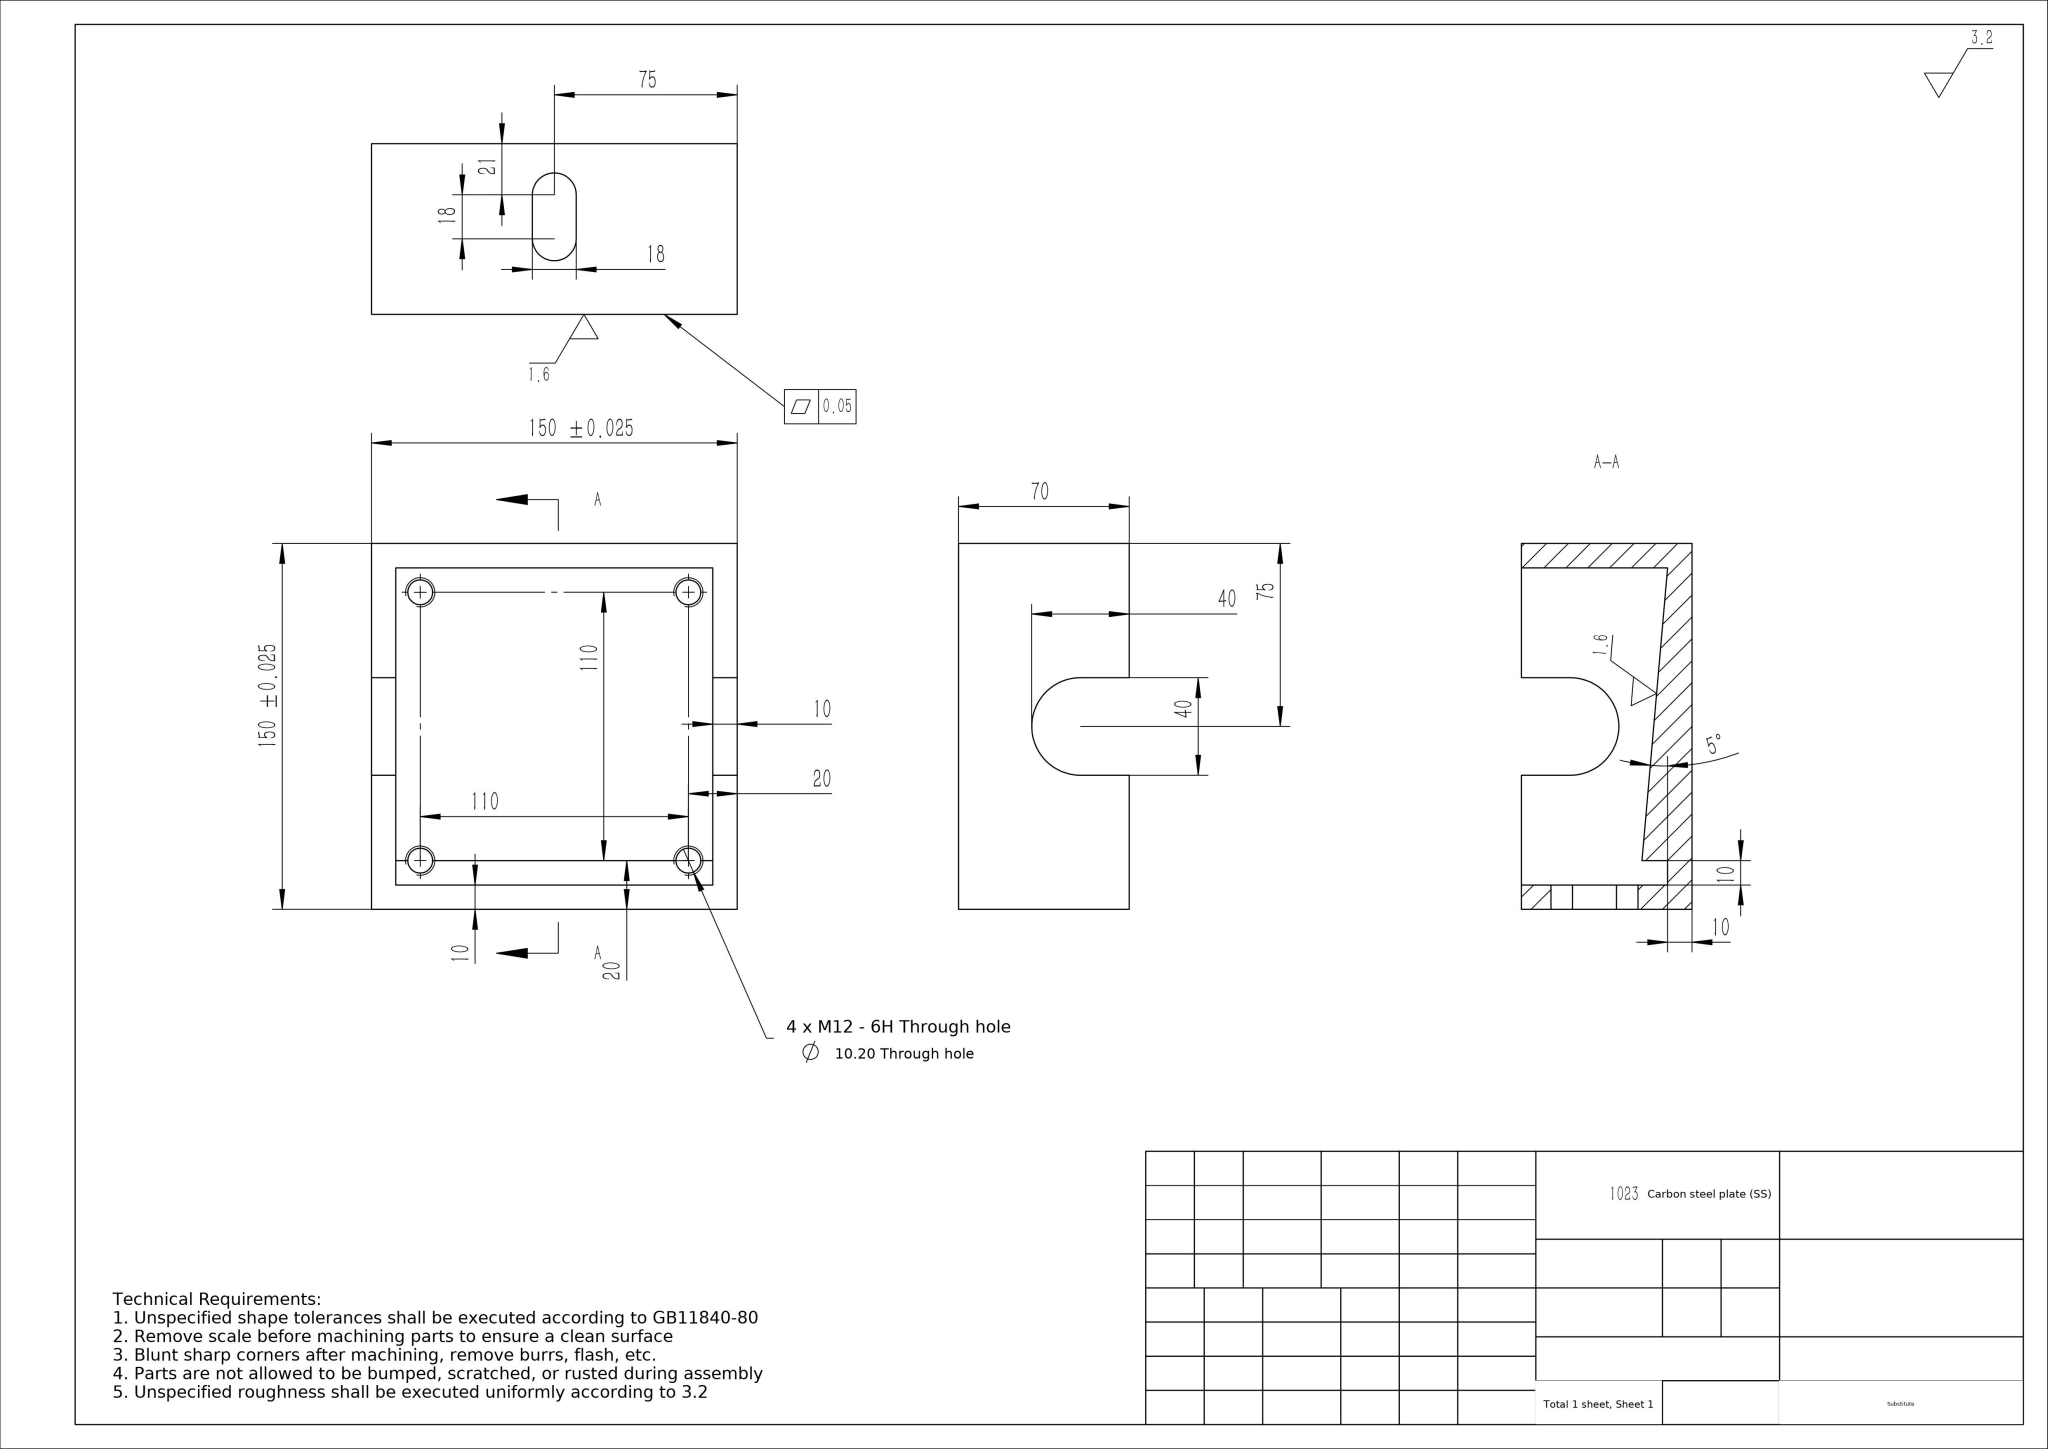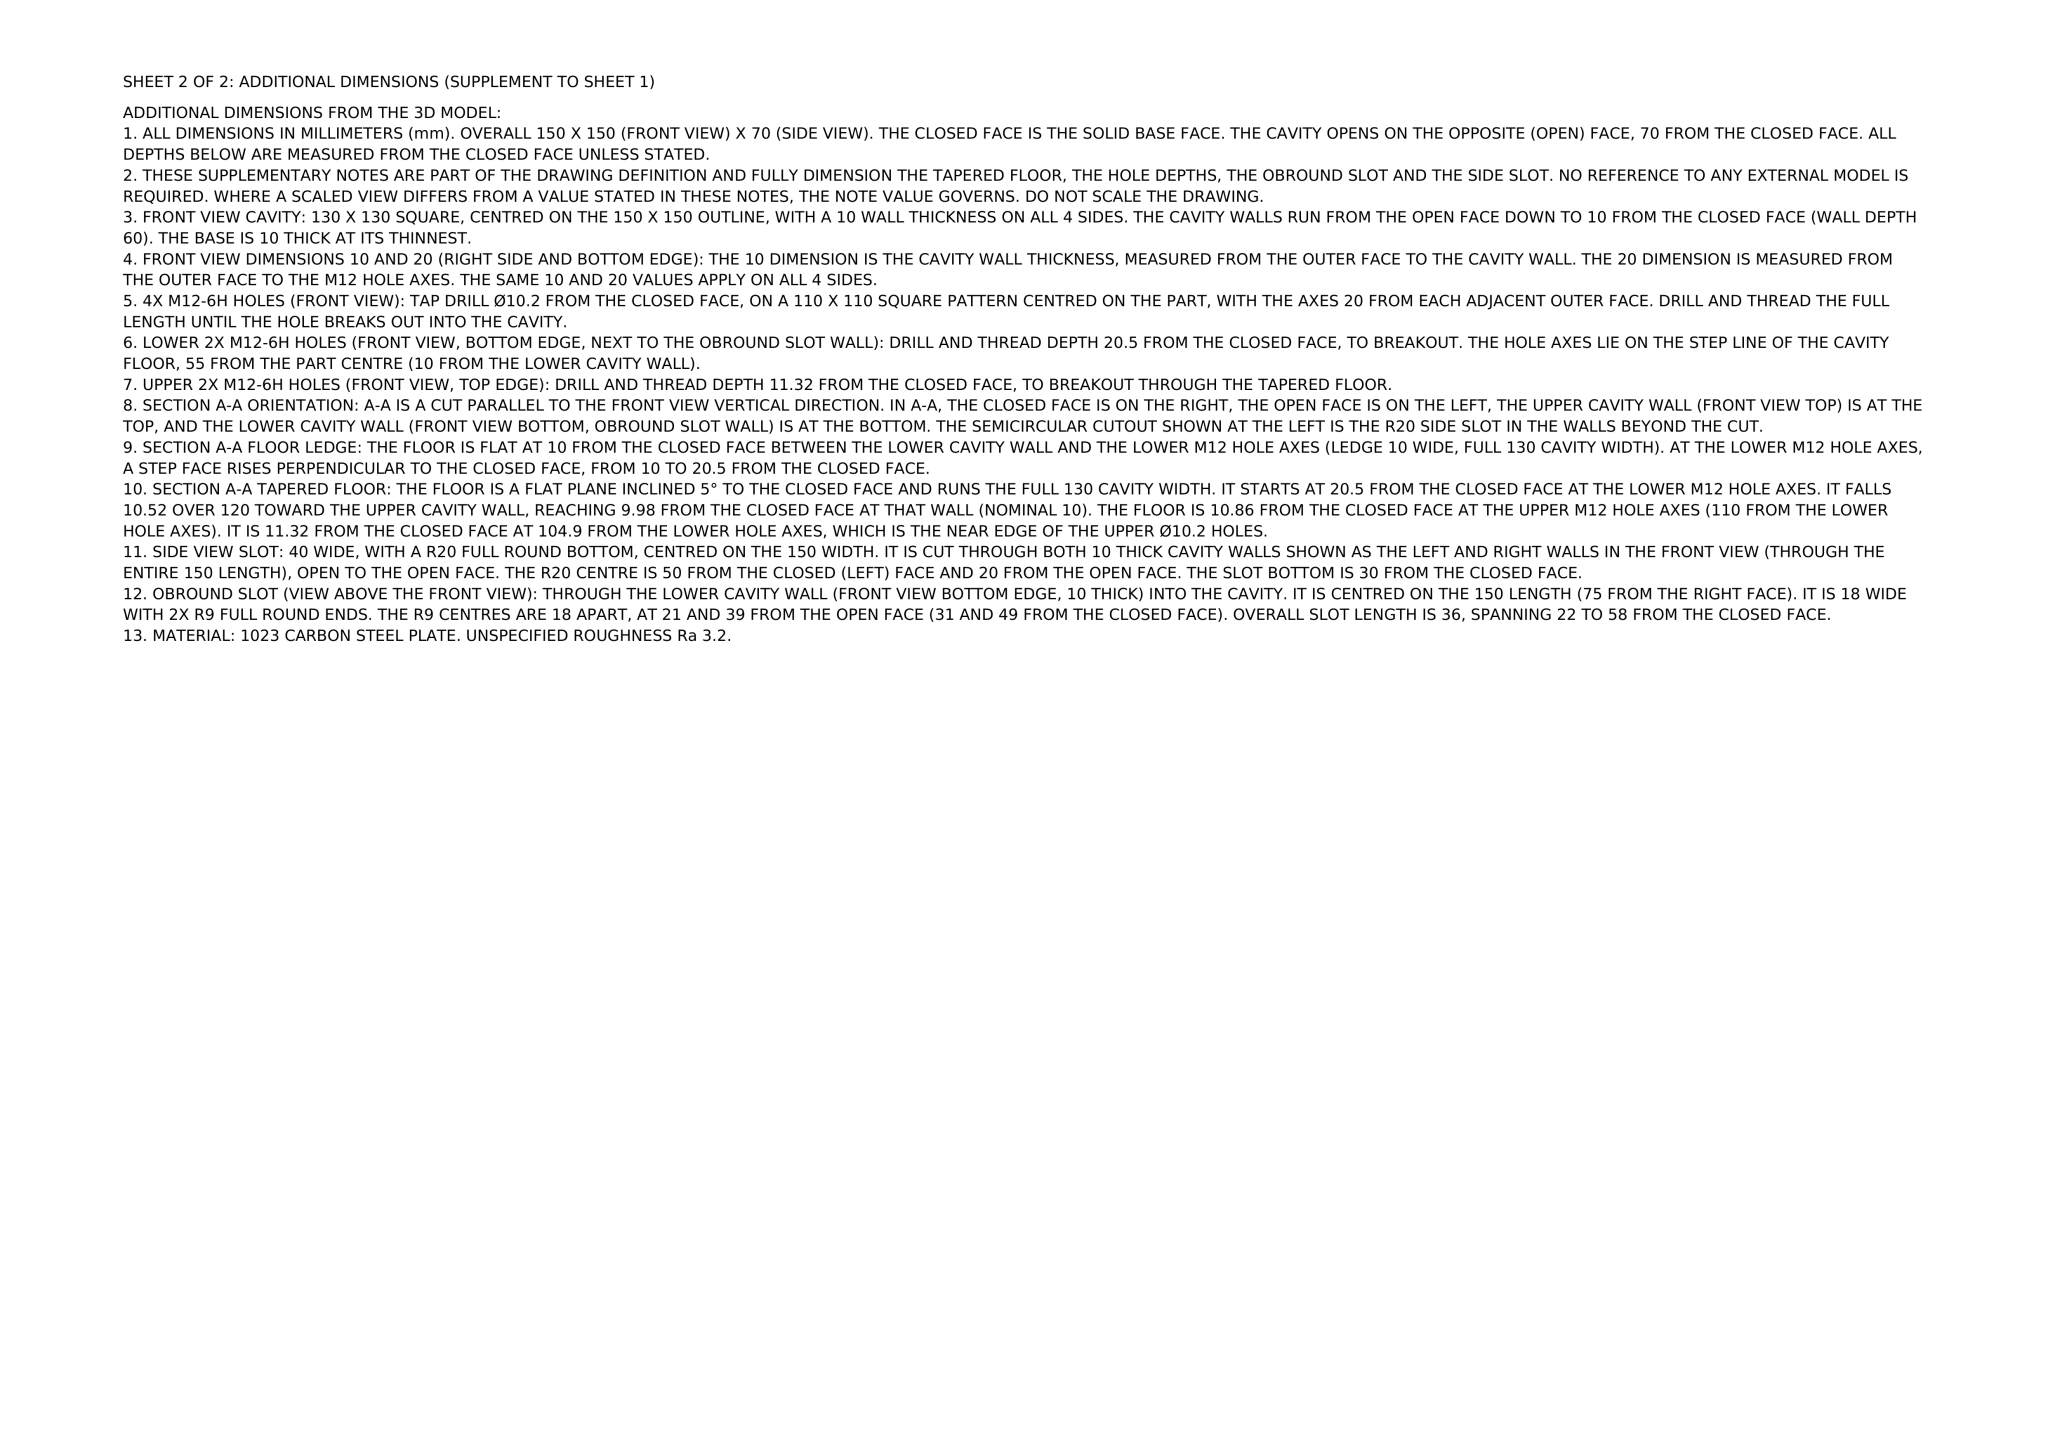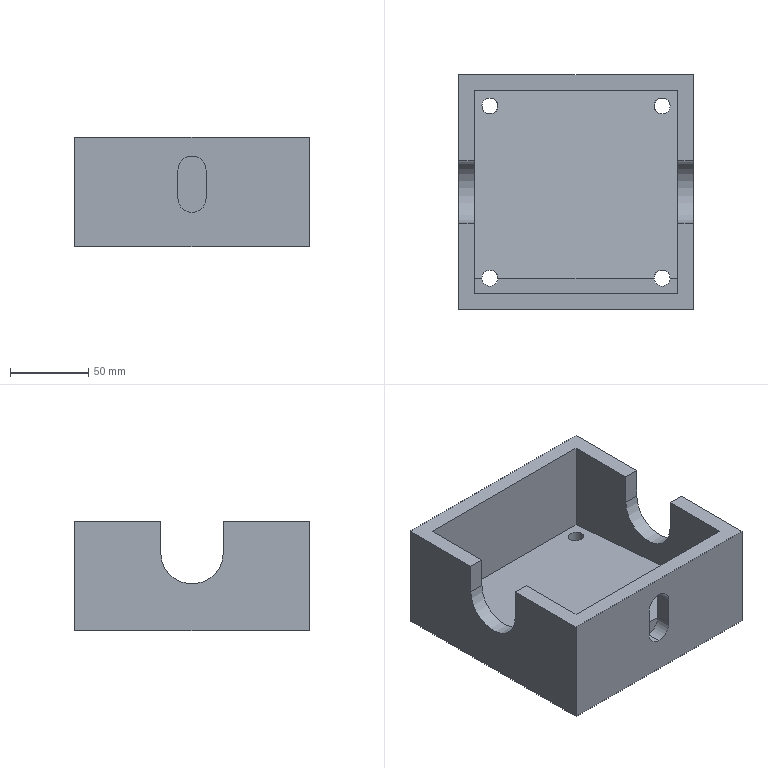Part | NX | mm | 1 solid | 35 faces | box 150 x 150 x 70 mm | volume 604284 mm3 | plane 22 | cylinder 13 | commonest cylinder face diameters 10.2 x8 18 x3 40 x2